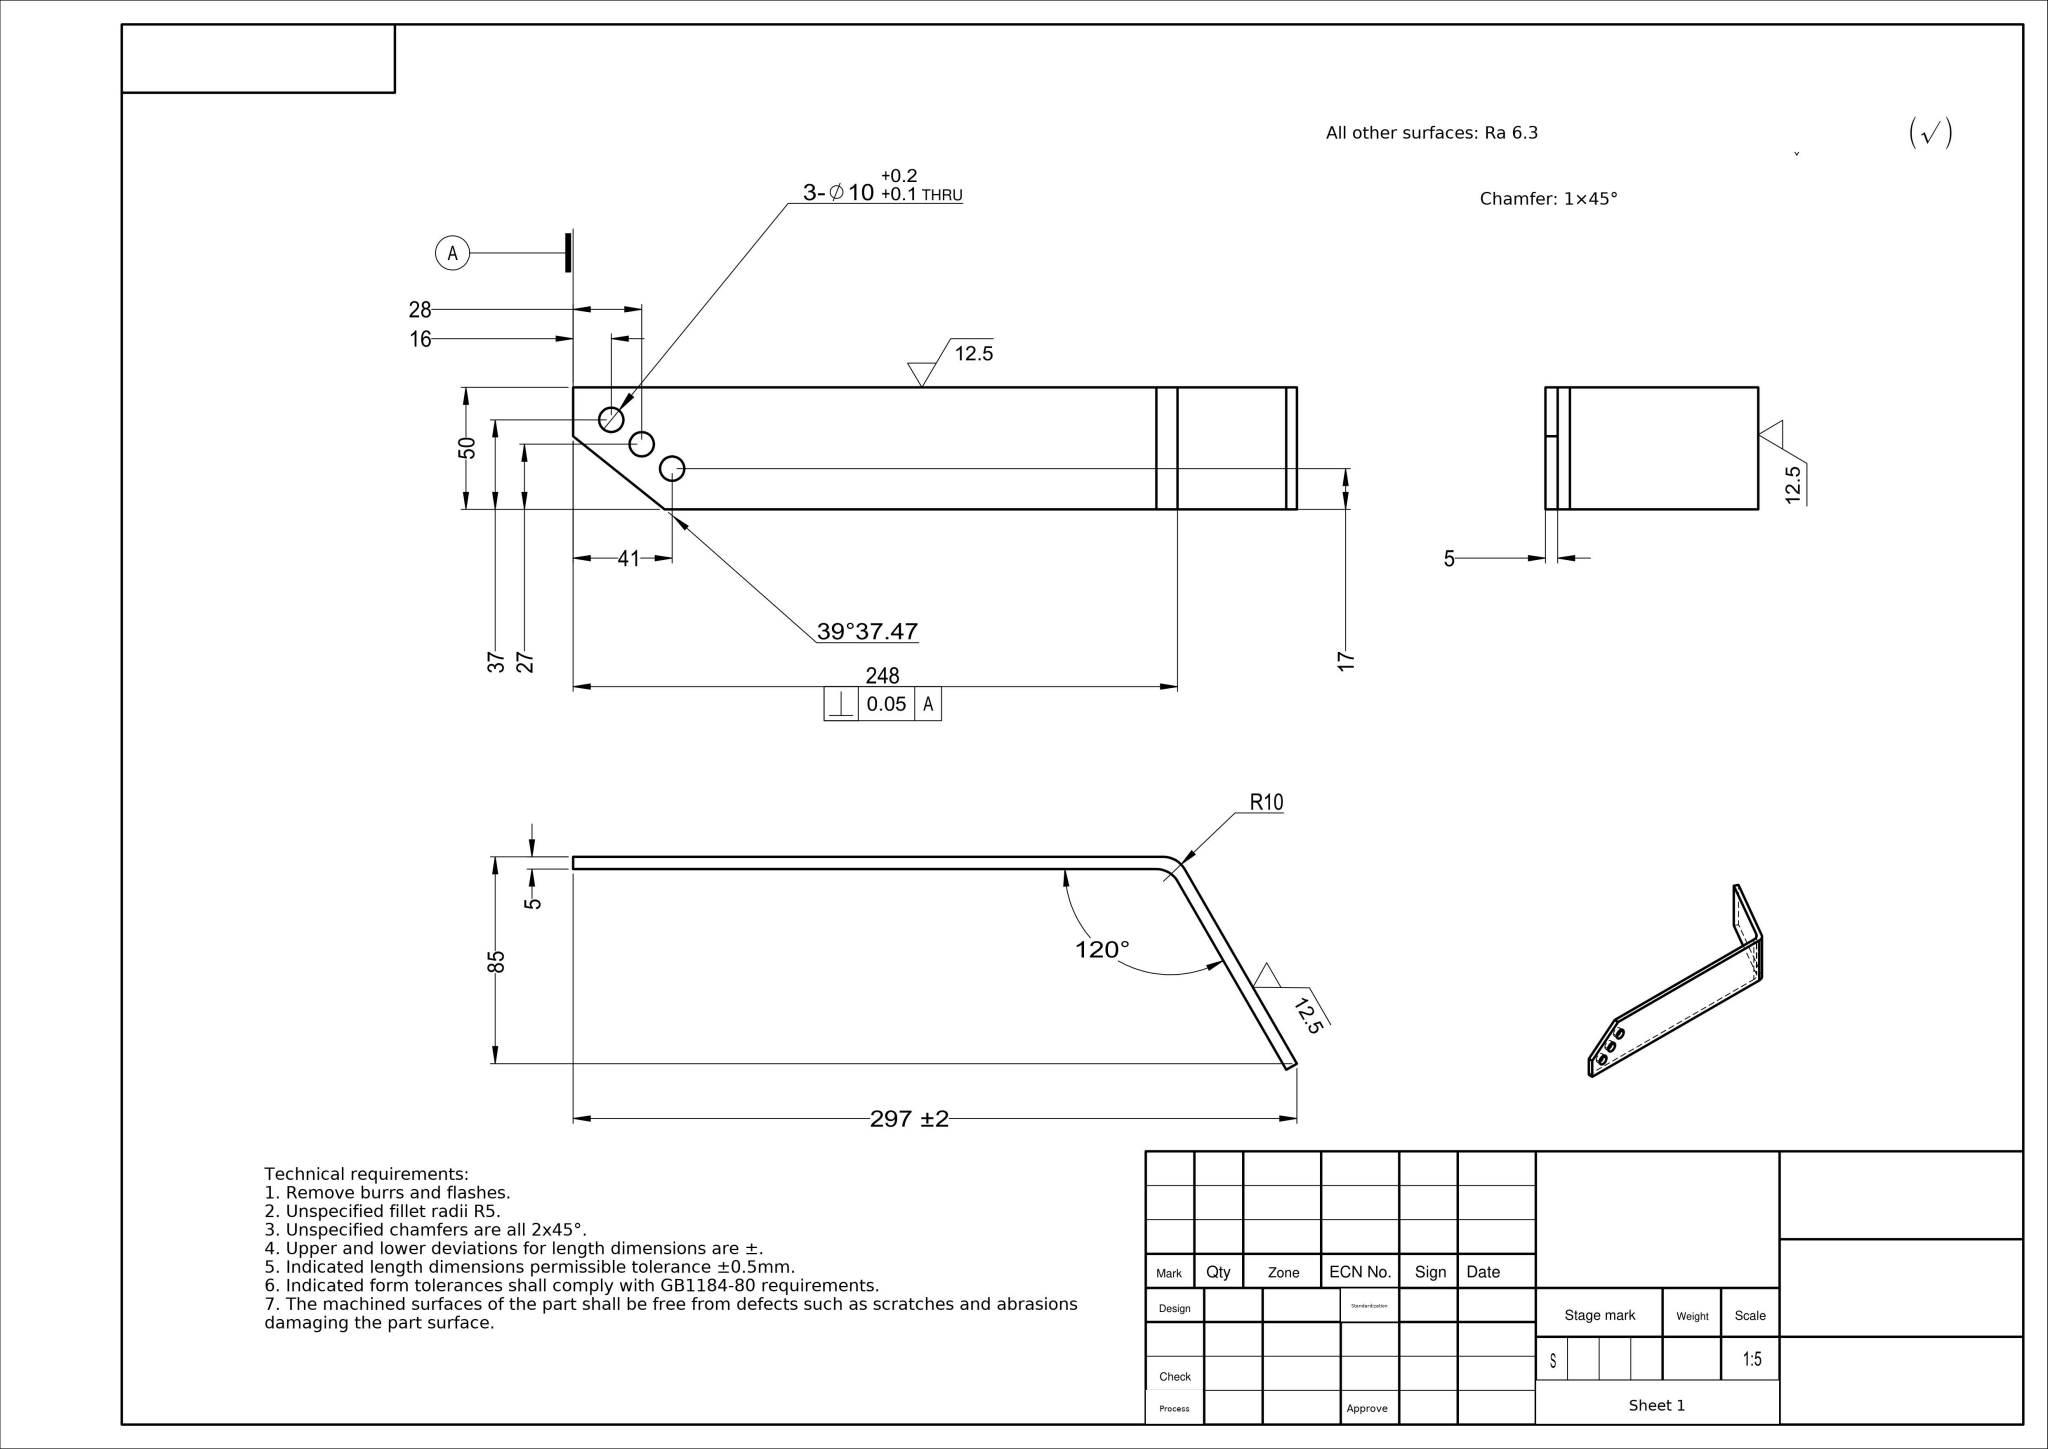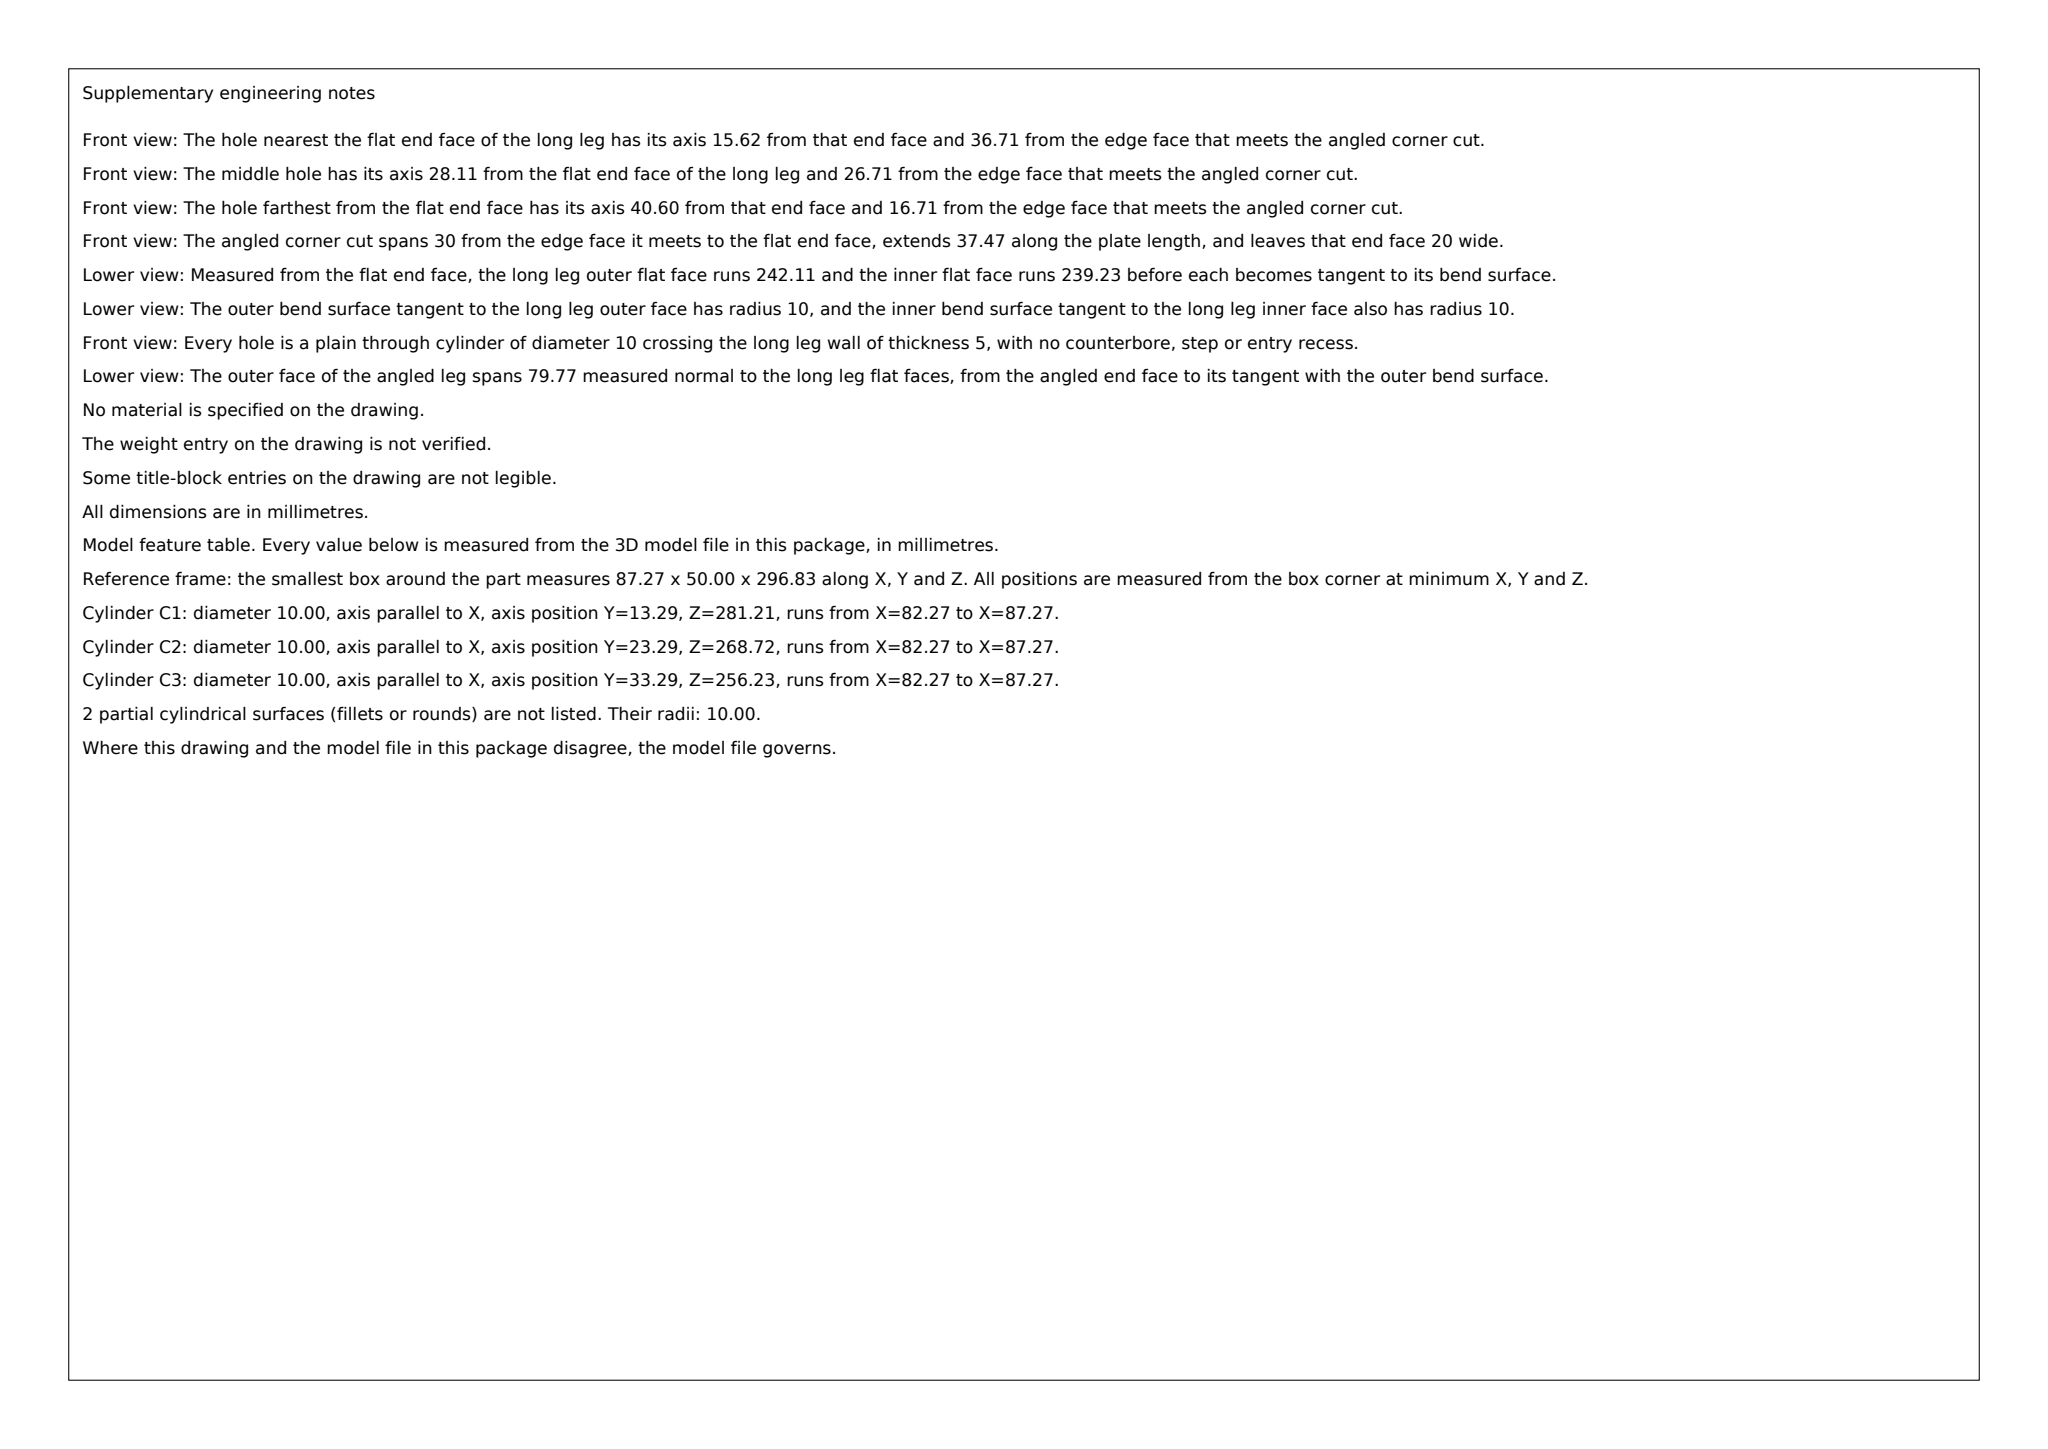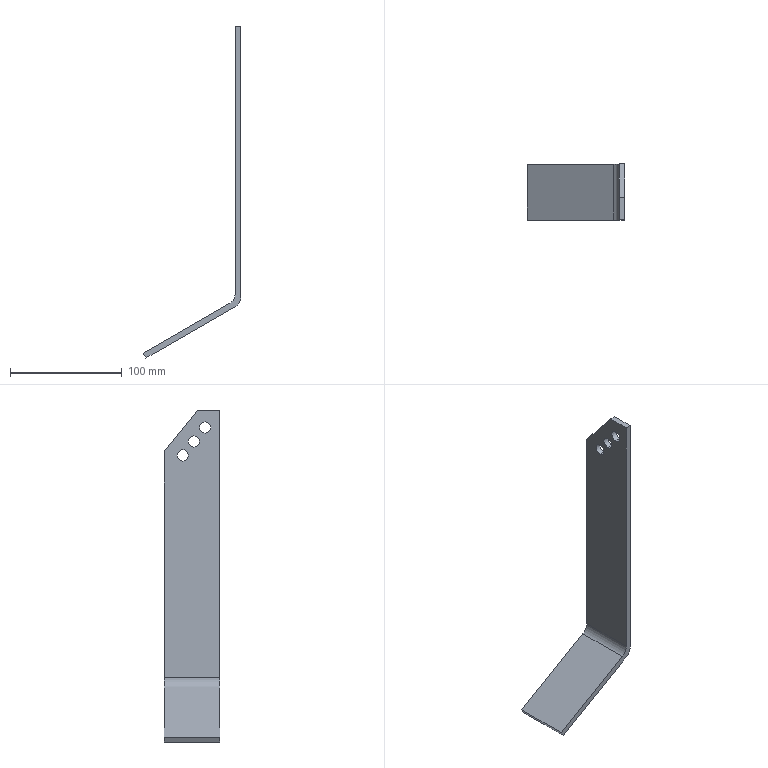Part | SolidWorks | mm | 1 solid | 17 faces | box 87.27 x 50 x 296.83 mm | volume 81733 mm3 | plane 9 | cylinder 8 | commonest cylinder face diameters 10 x6 20 x2
Drawing notes:
3X Ø10 (+0.2/+0.1) THRU holes in the 5 thick end flange, equally spaced 12.5 apart in the length direction; hole centers located 15.6, 28.1 and 40.6 from datum A (end face) | from the solid: cylinders[hole/bore, dia 10.0, axis x] at z = 281.2, 268.7, 256.2 with part end face at z = 296.8 (axis_planes z=296.8)
3X Ø10 hole centers also staggered 10 apart across the width: 13.3, 23.3 and 33.3 from the y=0 face | from the solid: cylinders[hole/bore, dia 10.0, axis x] at y = 13.3, 23.3, 33.3; axis_planes y=0.0
3X Ø10 (+0.2/+0.1) THRU holes equally spaced 12.5 apart in the length direction; hole centers at 15.6, 28.1 and 40.6 from datum A (end face). | from the solid: hole/bore Ø10 axis x at z=281.2, 268.7, 256.2 with end face plane z=296.8 (datum A); spacing 12.5, distances 15.6/28.1/40.6
STEP:
#1=CARTESIAN_POINT('',(77.272,50.,44.613));
#2=VERTEX_POINT('',#1);
#3=CARTESIAN_POINT('',(82.272,50.,53.274));
#4=VERTEX_POINT('',#3);
#5=CARTESIAN_POINT('',(72.272,50.,53.274));
#6=DIRECTION('',(0.,-1.,0.));
#7=DIRECTION('',(0.,0.,-1.));
#8=AXIS2_PLACEMENT_3D('',#5,#6,#7);
#9=CIRCLE('',#8,10.);
#10=EDGE_CURVE('',#2,#4,#9,.T.);
#11=ORIENTED_EDGE('',*,*,#10,.F.);
#12=CARTESIAN_POINT('',(77.272,0.,44.613));
#13=VERTEX_POINT('',#12);
#14=CARTESIAN_POINT('',(77.272,50.,44.613));
#15=DIRECTION('',(0.,1.,0.));
#16=VECTOR('',#15,1000.);
#17=LINE('',#14,#16);
#18=EDGE_CURVE('',#13,#2,#17,.T.);
#19=ORIENTED_EDGE('',*,*,#18,.F.);
#20=CARTESIAN_POINT('',(82.272,0.,53.274));
#21=VERTEX_POINT('',#20);
#22=CARTESIAN_POINT('',(72.272,0.,53.274));
#23=DIRECTION('',(0.,1.,0.));
#24=DIRECTION('',(0.,0.,-1.));
#25=AXIS2_PLACEMENT_3D('',#22,#23,#24);
#26=CIRCLE('',#25,10.);
#27=EDGE_CURVE('',#21,#13,#26,.T.);
#28=ORIENTED_EDGE('',*,*,#27,.F.);
#29=CARTESIAN_POINT('',(82.272,0.,53.274));
#30=DIRECTION('',(0.,-1.,0.));
#31=VECTOR('',#30,1000.);
#32=LINE('',#29,#31);
#33=EDGE_CURVE('',#4,#21,#32,.T.);
#34=ORIENTED_EDGE('',*,*,#33,.F.);
#35=EDGE_LOOP('',(#11,#19,#28,#34));
#36=FACE_OUTER_BOUND('',#35,.T.);
#37=CARTESIAN_POINT('',(72.272,50.,53.274));
#38=DIRECTION('',(0.,1.,0.));
#39=DIRECTION('',(0.,0.,1.));
#40=AXIS2_PLACEMENT_3D('',#37,#38,#39);
#41=CYLINDRICAL_SURFACE('',#40,10.);
#42=ADVANCED_FACE('',(#36),#41,.F.);
#43=CARTESIAN_POINT('',(87.272,50.,50.387));
#44=VERTEX_POINT('',#43);
#45=CARTESIAN_POINT('',(82.272,50.,41.726));
#46=VERTEX_POINT('',#45);
#47=CARTESIAN_POINT('',(77.272,50.,50.387));
#48=DIRECTION('',(0.,1.,0.));
#49=DIRECTION('',(0.,0.,-1.));
#50=AXIS2_PLACEMENT_3D('',#47,#48,#49);
#51=CIRCLE('',#50,10.);
#52=EDGE_CURVE('',#44,#46,#51,.T.);
#53=ORIENTED_EDGE('',*,*,#52,.F.);
#54=CARTESIAN_POINT('',(87.272,0.,50.387));
#55=VERTEX_POINT('',#54);
#56=CARTESIAN_POINT('',(87.272,50.,50.387));
#57=DIRECTION('',(0.,1.,0.));
#58=VECTOR('',#57,1000.);
#59=LINE('',#56,#58);
#60=EDGE_CURVE('',#55,#44,#59,.T.);
#61=ORIENTED_EDGE('',*,*,#60,.F.);
#62=CARTESIAN_POINT('',(82.272,0.,41.726));
#63=VERTEX_POINT('',#62);
#64=CARTESIAN_POINT('',(77.272,0.,50.387));
#65=DIRECTION('',(0.,-1.,0.));
#66=DIRECTION('',(0.,0.,-1.));
#67=AXIS2_PLACEMENT_3D('',#64,#65,#66);
#68=CIRCLE('',#67,10.);
#69=EDGE_CURVE('',#63,#55,#68,.T.);
#70=ORIENTED_EDGE('',*,*,#69,.F.);
#71=CARTESIAN_POINT('',(82.272,50.,41.726));
#72=DIRECTION('',(0.,-1.,0.));
#73=VECTOR('',#72,1000.);
#74=LINE('',#71,#73);
#75=EDGE_CURVE('',#46,#63,#74,.T.);
#76=ORIENTED_EDGE('',*,*,#75,.F.);
#77=EDGE_LOOP('',(#53,#61,#70,#76));
#78=FACE_OUTER_BOUND('',#77,.T.);
#79=CARTESIAN_POINT('',(77.272,50.,50.387));
#80=DIRECTION('',(0.,-1.,0.));
#81=DIRECTION('',(0.,0.,-1.));
#82=AXIS2_PLACEMENT_3D('',#79,#80,#81);
#83=CYLINDRICAL_SURFACE('',#82,10.);
#84=ADVANCED_FACE('',(#78),#83,.T.);
#85=CARTESIAN_POINT('',(82.272,13.291,281.88));
#86=VERTEX_POINT('',#85);
#87=CARTESIAN_POINT('',(87.272,13.291,281.88));
#88=VERTEX_POINT('',#87);
#89=CARTESIAN_POINT('',(37.272,13.291,281.88));
#90=DIRECTION('',(1.,0.,0.));
#91=VECTOR('',#90,1000.);
#92=LINE('',#89,#91);
#93=EDGE_CURVE('',#86,#88,#92,.T.);
#94=ORIENTED_EDGE('',*,*,#93,.F.);
#95=CARTESIAN_POINT('',(82.272,13.291,271.88));
#96=VERTEX_POINT('',#95);
#97=CARTESIAN_POINT('',(82.272,13.291,276.88));
#98=DIRECTION('',(1.,0.,0.));
#99=DIRECTION('',(0.,0.,-1.));
#100=AXIS2_PLACEMENT_3D('',#97,#98,#99);
#101=CIRCLE('',#100,5.);
#102=EDGE_CURVE('',#96,#86,#101,.T.);
#103=ORIENTED_EDGE('',*,*,#102,.F.);
#104=CARTESIAN_POINT('',(87.272,13.291,271.88));
#105=VERTEX_POINT('',#104);
#106=CARTESIAN_POINT('',(37.272,13.291,271.88));
#107=DIRECTION('',(1.,0.,0.));
#108=VECTOR('',#107,1000.);
#109=LINE('',#106,#108);
#110=EDGE_CURVE('',#96,#105,#109,.T.);
#111=ORIENTED_EDGE('',*,*,#110,.T.);
#112=CARTESIAN_POINT('',(87.272,13.291,276.88));
#113=DIRECTION('',(1.,0.,0.));
#114=DIRECTION('',(0.,0.,-1.));
#115=AXIS2_PLACEMENT_3D('',#112,#113,#114);
#116=CIRCLE('',#115,5.);
#117=EDGE_CURVE('',#105,#88,#116,.T.);
#118=ORIENTED_EDGE('',*,*,#117,.T.);
#119=EDGE_LOOP('',(#94,#103,#111,#118));
#120=FACE_OUTER_BOUND('',#119,.T.);
#121=CARTESIAN_POINT('',(37.272,13.291,276.88));
#122=DIRECTION('',(1.,0.,0.));
#123=DIRECTION('',(0.,0.,-1.));
#124=AXIS2_PLACEMENT_3D('',#121,#122,#123);
#125=CYLINDRICAL_SURFACE('',#124,5.);
#126=ADVANCED_FACE('',(#120),#125,.F.);
#127=CARTESIAN_POINT('',(82.272,33.291,256.9));
#128=VERTEX_POINT('',#127);
#129=CARTESIAN_POINT('',(87.272,33.291,256.9));
#130=VERTEX_POINT('',#129);
#131=CARTESIAN_POINT('',(37.272,33.291,256.9));
#132=DIRECTION('',(1.,0.,0.));
#133=VECTOR('',#132,1000.);
#134=LINE('',#131,#133);
#135=EDGE_CURVE('',#128,#130,#134,.T.);
#136=ORIENTED_EDGE('',*,*,#135,.F.);
#137=CARTESIAN_POINT('',(82.272,33.291,246.9));
#138=VERTEX_POINT('',#137);
#139=CARTESIAN_POINT('',(82.272,33.291,251.9));
#140=DIRECTION('',(1.,0.,0.));
#141=DIRECTION('',(0.,0.,-1.));
#142=AXIS2_PLACEMENT_3D('',#139,#140,#141);
#143=CIRCLE('',#142,5.);
#144=EDGE_CURVE('',#138,#128,#143,.T.);
#145=ORIENTED_EDGE('',*,*,#144,.F.);
#146=CARTESIAN_POINT('',(87.272,33.291,246.9));
#147=VERTEX_POINT('',#146);
#148=CARTESIAN_POINT('',(37.272,33.291,246.9));
#149=DIRECTION('',(1.,0.,0.));
#150=VECTOR('',#149,1000.);
#151=LINE('',#148,#150);
#152=EDGE_CURVE('',#138,#147,#151,.T.);
#153=ORIENTED_EDGE('',*,*,#152,.T.);
#154=CARTESIAN_POINT('',(87.272,33.291,251.9));
#155=DIRECTION('',(1.,0.,0.));
#156=DIRECTION('',(0.,0.,-1.));
#157=AXIS2_PLACEMENT_3D('',#154,#155,#156);
#158=CIRCLE('',#157,5.);
#159=EDGE_CURVE('',#147,#130,#158,.T.);
#160=ORIENTED_EDGE('',*,*,#159,.T.);
#161=EDGE_LOOP('',(#136,#145,#153,#160));
#162=FACE_OUTER_BOUND('',#161,.T.);
#163=CARTESIAN_POINT('',(37.272,33.291,251.9));
#164=DIRECTION('',(1.,0.,0.));
#165=DIRECTION('',(0.,0.,-1.));
#166=AXIS2_PLACEMENT_3D('',#163,#164,#165);
#167=CYLINDRICAL_SURFACE('',#166,5.);
#168=ADVANCED_FACE('',(#162),#167,.F.);
#169=CARTESIAN_POINT('',(82.272,23.291,269.39));
#170=VERTEX_POINT('',#169);
#171=CARTESIAN_POINT('',(87.272,23.291,269.39));
#172=VERTEX_POINT('',#171);
#173=CARTESIAN_POINT('',(37.272,23.291,269.39));
#174=DIRECTION('',(1.,0.,0.));
#175=VECTOR('',#174,1000.);
#176=LINE('',#173,#175);
#177=EDGE_CURVE('',#170,#172,#176,.T.);
#178=ORIENTED_EDGE('',*,*,#177,.F.);
#179=CARTESIAN_POINT('',(82.272,23.291,259.39));
#180=VERTEX_POINT('',#179);
#181=CARTESIAN_POINT('',(82.272,23.291,264.39));
#182=DIRECTION('',(1.,0.,0.));
#183=DIRECTION('',(0.,0.,-1.));
#184=AXIS2_PLACEMENT_3D('',#181,#182,#183);
#185=CIRCLE('',#184,5.);
#186=EDGE_CURVE('',#180,#170,#185,.T.);
#187=ORIENTED_EDGE('',*,*,#186,.F.);
#188=CARTESIAN_POINT('',(87.272,23.291,259.39));
#189=VERTEX_POINT('',#188);
#190=CARTESIAN_POINT('',(37.272,23.291,259.39));
#191=DIRECTION('',(1.,0.,0.));
#192=VECTOR('',#191,1000.);
#193=LINE('',#190,#192);
#194=EDGE_CURVE('',#180,#189,#193,.T.);
#195=ORIENTED_EDGE('',*,*,#194,.T.);
#196=CARTESIAN_POINT('',(87.272,23.291,264.39));
#197=DIRECTION('',(1.,0.,0.));
#198=DIRECTION('',(0.,0.,-1.));
#199=AXIS2_PLACEMENT_3D('',#196,#197,#198);
#200=CIRCLE('',#199,5.);
#201=EDGE_CURVE('',#189,#172,#200,.T.);
#202=ORIENTED_EDGE('',*,*,#201,.T.);
#203=EDGE_LOOP('',(#178,#187,#195,#202));
#204=FACE_OUTER_BOUND('',#203,.T.);
#205=CARTESIAN_POINT('',(37.272,23.291,264.39));
#206=DIRECTION('',(1.,0.,0.));
#207=DIRECTION('',(0.,0.,-1.));
#208=AXIS2_PLACEMENT_3D('',#205,#206,#207);
#209=CYLINDRICAL_SURFACE('',#208,5.);
#210=ADVANCED_FACE('',(#204),#209,.F.);
#211=CARTESIAN_POINT('',(82.272,20.,292.5));
#212=VERTEX_POINT('',#211);
#213=CARTESIAN_POINT('',(87.272,20.,292.5));
#214=VERTEX_POINT('',#213);
#215=CARTESIAN_POINT('',(37.272,20.,292.5));
#216=DIRECTION('',(1.,0.,0.));
#217=VECTOR('',#216,1000.);
#218=LINE('',#215,#217);
#219=EDGE_CURVE('',#212,#214,#218,.T.);
#220=ORIENTED_EDGE('',*,*,#219,.T.);
#221=CARTESIAN_POINT('',(87.272,50.,255.03));
#222=VERTEX_POINT('',#221);
#223=CARTESIAN_POINT('',(87.272,50.,255.03));
#224=DIRECTION('',(0.,0.625,-0.7806));
#225=VECTOR('',#224,1000.);
#226=LINE('',#223,#225);
#227=EDGE_CURVE('',#214,#222,#226,.T.);
#228=ORIENTED_EDGE('',*,*,#227,.T.);
#229=CARTESIAN_POINT('',(82.272,50.,255.03));
#230=VERTEX_POINT('',#229);
#231=CARTESIAN_POINT('',(0.,50.,255.03));
#232=DIRECTION('',(1.,0.,0.));
#233=VECTOR('',#232,1000.);
#234=LINE('',#231,#233);
#235=EDGE_CURVE('',#230,#222,#234,.T.);
#236=ORIENTED_EDGE('',*,*,#235,.F.);
#237=CARTESIAN_POINT('',(82.272,151.252,128.566));
#238=DIRECTION('',(-0.,0.625,-0.7806));
#239=VECTOR('',#238,1000.);
#240=LINE('',#237,#239);
#241=EDGE_CURVE('',#212,#230,#240,.T.);
#242=ORIENTED_EDGE('',*,*,#241,.F.);
#243=EDGE_LOOP('',(#220,#228,#236,#242));
#244=FACE_OUTER_BOUND('',#243,.T.);
#245=CARTESIAN_POINT('',(37.272,50.,255.03));
#246=DIRECTION('',(0.,-0.7806,-0.625));
#247=DIRECTION('',(0.,0.625,-0.7806));
#248=AXIS2_PLACEMENT_3D('',#245,#246,#247);
#249=PLANE('',#248);
#250=ADVANCED_FACE('',(#244),#249,.F.);
#251=CARTESIAN_POINT('',(2.5,0.,-4.33));
#252=VERTEX_POINT('',#251);
#253=CARTESIAN_POINT('',(2.5,0.,-4.33));
#254=DIRECTION('',(-0.866,0.,-0.5));
#255=VECTOR('',#254,1000.);
#256=LINE('',#253,#255);
#257=EDGE_CURVE('',#63,#252,#256,.T.);
#258=ORIENTED_EDGE('',*,*,#257,.F.);
#259=ORIENTED_EDGE('',*,*,#69,.T.);
#260=CARTESIAN_POINT('',(87.272,0.,292.5));
#261=VERTEX_POINT('',#260);
#262=CARTESIAN_POINT('',(87.272,0.,44.613));
#263=DIRECTION('',(-0.,0.,-1.));
#264=VECTOR('',#263,1000.);
#265=LINE('',#262,#264);
#266=EDGE_CURVE('',#261,#55,#265,.T.);
#267=ORIENTED_EDGE('',*,*,#266,.F.);
#268=CARTESIAN_POINT('',(82.272,0.,292.5));
#269=VERTEX_POINT('',#268);
#270=CARTESIAN_POINT('',(82.272,0.,292.5));
#271=DIRECTION('',(1.,0.,0.));
#272=VECTOR('',#271,1000.);
#273=LINE('',#270,#272);
#274=EDGE_CURVE('',#269,#261,#273,.T.);
#275=ORIENTED_EDGE('',*,*,#274,.F.);
#276=CARTESIAN_POINT('',(82.272,0.,47.5));
#277=DIRECTION('',(0.,0.,1.));
#278=VECTOR('',#277,1000.);
#279=LINE('',#276,#278);
#280=EDGE_CURVE('',#21,#269,#279,.T.);
#281=ORIENTED_EDGE('',*,*,#280,.F.);
#282=ORIENTED_EDGE('',*,*,#27,.T.);
#283=CARTESIAN_POINT('',(0.,0.,0.));
#284=VERTEX_POINT('',#283);
#285=CARTESIAN_POINT('',(0.,0.,0.));
#286=DIRECTION('',(0.866,0.,0.5));
#287=VECTOR('',#286,1000.);
#288=LINE('',#285,#287);
#289=EDGE_CURVE('',#284,#13,#288,.T.);
#290=ORIENTED_EDGE('',*,*,#289,.F.);
#291=CARTESIAN_POINT('',(0.,0.,0.));
#292=DIRECTION('',(-0.5,0.,0.866));
#293=VECTOR('',#292,1000.);
#294=LINE('',#291,#293);
#295=EDGE_CURVE('',#252,#284,#294,.T.);
#296=ORIENTED_EDGE('',*,*,#295,.F.);
#297=EDGE_LOOP('',(#258,#259,#267,#275,#281,#282,#290,#296));
#298=FACE_OUTER_BOUND('',#297,.T.);
#299=CARTESIAN_POINT('',(0.,0.,0.));
#300=DIRECTION('',(0.,-1.,0.));
#301=DIRECTION('',(0.,0.,-1.));
#302=AXIS2_PLACEMENT_3D('',#299,#300,#301);
#303=PLANE('',#302);
#304=ADVANCED_FACE('',(#298),#303,.T.);
#305=CARTESIAN_POINT('',(87.272,50.,44.613));
#306=DIRECTION('',(-0.,0.,-1.));
#307=VECTOR('',#306,1000.);
#308=LINE('',#305,#307);
#309=EDGE_CURVE('',#222,#44,#308,.T.);
#310=ORIENTED_EDGE('',*,*,#309,.T.);
#311=ORIENTED_EDGE('',*,*,#52,.T.);
#312=CARTESIAN_POINT('',(2.5,50.,-4.33));
#313=VERTEX_POINT('',#312);
#314=CARTESIAN_POINT('',(2.5,50.,-4.33));
#315=DIRECTION('',(-0.866,0.,-0.5));
#316=VECTOR('',#315,1000.);
#317=LINE('',#314,#316);
#318=EDGE_CURVE('',#46,#313,#317,.T.);
#319=ORIENTED_EDGE('',*,*,#318,.T.);
#320=CARTESIAN_POINT('',(0.,50.,0.));
#321=VERTEX_POINT('',#320);
#322=CARTESIAN_POINT('',(0.,50.,0.));
#323=DIRECTION('',(-0.5,0.,0.866));
#324=VECTOR('',#323,1000.);
#325=LINE('',#322,#324);
#326=EDGE_CURVE('',#313,#321,#325,.T.);
#327=ORIENTED_EDGE('',*,*,#326,.T.);
#328=CARTESIAN_POINT('',(0.,50.,0.));
#329=DIRECTION('',(0.866,0.,0.5));
#330=VECTOR('',#329,1000.);
#331=LINE('',#328,#330);
#332=EDGE_CURVE('',#321,#2,#331,.T.);
#333=ORIENTED_EDGE('',*,*,#332,.T.);
#334=ORIENTED_EDGE('',*,*,#10,.T.);
#335=CARTESIAN_POINT('',(82.272,50.,47.5));
#336=DIRECTION('',(0.,0.,1.));
#337=VECTOR('',#336,1000.);
#338=LINE('',#335,#337);
#339=EDGE_CURVE('',#4,#230,#338,.T.);
#340=ORIENTED_EDGE('',*,*,#339,.T.);
#341=ORIENTED_EDGE('',*,*,#235,.T.);
#342=EDGE_LOOP('',(#310,#311,#319,#327,#333,#334,#340,#341));
#343=FACE_OUTER_BOUND('',#342,.T.);
#344=CARTESIAN_POINT('',(0.,50.,0.));
#345=DIRECTION('',(0.,-1.,0.));
#346=DIRECTION('',(0.,0.,-1.));
#347=AXIS2_PLACEMENT_3D('',#344,#345,#346);
#348=PLANE('',#347);
#349=ADVANCED_FACE('',(#343),#348,.F.);
#350=ORIENTED_EDGE('',*,*,#318,.F.);
#351=ORIENTED_EDGE('',*,*,#75,.T.);
#352=ORIENTED_EDGE('',*,*,#257,.T.);
#353=CARTESIAN_POINT('',(2.5,50.,-4.33));
#354=DIRECTION('',(0.,-1.,0.));
#355=VECTOR('',#354,1000.);
#356=LINE('',#353,#355);
#357=EDGE_CURVE('',#313,#252,#356,.T.);
#358=ORIENTED_EDGE('',*,*,#357,.F.);
#359=EDGE_LOOP('',(#350,#351,#352,#358));
#360=FACE_OUTER_BOUND('',#359,.T.);
#361=CARTESIAN_POINT('',(2.5,50.,-4.33));
#362=DIRECTION('',(-0.5,0.,0.866));
#363=DIRECTION('',(0.,1.,0.));
#364=AXIS2_PLACEMENT_3D('',#361,#362,#363);
#365=PLANE('',#364);
#366=ADVANCED_FACE('',(#360),#365,.F.);
#367=ORIENTED_EDGE('',*,*,#201,.F.);
#368=CARTESIAN_POINT('',(87.272,23.291,264.39));
#369=DIRECTION('',(1.,0.,0.));
#370=DIRECTION('',(0.,0.,-1.));
#371=AXIS2_PLACEMENT_3D('',#368,#369,#370);
#372=CIRCLE('',#371,5.);
#373=EDGE_CURVE('',#172,#189,#372,.T.);
#374=ORIENTED_EDGE('',*,*,#373,.F.);
#375=EDGE_LOOP('',(#367,#374));
#376=FACE_BOUND('',#375,.T.);
#377=ORIENTED_EDGE('',*,*,#159,.F.);
#378=CARTESIAN_POINT('',(87.272,33.291,251.9));
#379=DIRECTION('',(1.,0.,0.));
#380=DIRECTION('',(0.,0.,-1.));
#381=AXIS2_PLACEMENT_3D('',#378,#379,#380);
#382=CIRCLE('',#381,5.);
#383=EDGE_CURVE('',#130,#147,#382,.T.);
#384=ORIENTED_EDGE('',*,*,#383,.F.);
#385=EDGE_LOOP('',(#377,#384));
#386=FACE_BOUND('',#385,.T.);
#387=ORIENTED_EDGE('',*,*,#117,.F.);
#388=CARTESIAN_POINT('',(87.272,13.291,276.88));
#389=DIRECTION('',(1.,0.,0.));
#390=DIRECTION('',(0.,0.,-1.));
#391=AXIS2_PLACEMENT_3D('',#388,#389,#390);
#392=CIRCLE('',#391,5.);
#393=EDGE_CURVE('',#88,#105,#392,.T.);
#394=ORIENTED_EDGE('',*,*,#393,.F.);
#395=EDGE_LOOP('',(#387,#394));
#396=FACE_BOUND('',#395,.T.);
#397=ORIENTED_EDGE('',*,*,#266,.T.);
#398=ORIENTED_EDGE('',*,*,#60,.T.);
#399=ORIENTED_EDGE('',*,*,#309,.F.);
#400=ORIENTED_EDGE('',*,*,#227,.F.);
#401=CARTESIAN_POINT('',(87.272,50.,292.5));
#402=DIRECTION('',(0.,-1.,0.));
#403=VECTOR('',#402,1000.);
#404=LINE('',#401,#403);
#405=EDGE_CURVE('',#214,#261,#404,.T.);
#406=ORIENTED_EDGE('',*,*,#405,.T.);
#407=EDGE_LOOP('',(#397,#398,#399,#400,#406));
#408=FACE_OUTER_BOUND('',#407,.T.);
#409=CARTESIAN_POINT('',(87.272,50.,44.613));
#410=DIRECTION('',(-1.,0.,0.));
#411=DIRECTION('',(0.,1.,0.));
#412=AXIS2_PLACEMENT_3D('',#409,#410,#411);
#413=PLANE('',#412);
#414=ADVANCED_FACE('',(#376,#386,#396,#408),#413,.F.);
#415=ORIENTED_EDGE('',*,*,#405,.F.);
#416=ORIENTED_EDGE('',*,*,#219,.F.);
#417=CARTESIAN_POINT('',(82.272,50.,292.5));
#418=DIRECTION('',(0.,-1.,0.));
#419=VECTOR('',#418,1000.);
#420=LINE('',#417,#419);
#421=EDGE_CURVE('',#212,#269,#420,.T.);
#422=ORIENTED_EDGE('',*,*,#421,.T.);
#423=ORIENTED_EDGE('',*,*,#274,.T.);
#424=EDGE_LOOP('',(#415,#416,#422,#423));
#425=FACE_OUTER_BOUND('',#424,.T.);
#426=CARTESIAN_POINT('',(82.272,50.,292.5));
#427=DIRECTION('',(0.,0.,-1.));
#428=DIRECTION('',(0.,-1.,0.));
#429=AXIS2_PLACEMENT_3D('',#426,#427,#428);
#430=PLANE('',#429);
#431=ADVANCED_FACE('',(#425),#430,.F.);
#432=ORIENTED_EDGE('',*,*,#186,.T.);
#433=CARTESIAN_POINT('',(82.272,23.291,264.39));
#434=DIRECTION('',(1.,0.,0.));
#435=DIRECTION('',(0.,0.,-1.));
#436=AXIS2_PLACEMENT_3D('',#433,#434,#435);
#437=CIRCLE('',#436,5.);
#438=EDGE_CURVE('',#170,#180,#437,.T.);
#439=ORIENTED_EDGE('',*,*,#438,.T.);
#440=EDGE_LOOP('',(#432,#439));
#441=FACE_BOUND('',#440,.T.);
#442=ORIENTED_EDGE('',*,*,#144,.T.);
#443=CARTESIAN_POINT('',(82.272,33.291,251.9));
#444=DIRECTION('',(1.,0.,0.));
#445=DIRECTION('',(0.,0.,-1.));
#446=AXIS2_PLACEMENT_3D('',#443,#444,#445);
#447=CIRCLE('',#446,5.);
#448=EDGE_CURVE('',#128,#138,#447,.T.);
#449=ORIENTED_EDGE('',*,*,#448,.T.);
#450=EDGE_LOOP('',(#442,#449));
#451=FACE_BOUND('',#450,.T.);
#452=ORIENTED_EDGE('',*,*,#102,.T.);
#453=CARTESIAN_POINT('',(82.272,13.291,276.88));
#454=DIRECTION('',(1.,0.,0.));
#455=DIRECTION('',(0.,0.,-1.));
#456=AXIS2_PLACEMENT_3D('',#453,#454,#455);
#457=CIRCLE('',#456,5.);
#458=EDGE_CURVE('',#86,#96,#457,.T.);
#459=ORIENTED_EDGE('',*,*,#458,.T.);
#460=EDGE_LOOP('',(#452,#459));
#461=FACE_BOUND('',#460,.T.);
#462=ORIENTED_EDGE('',*,*,#339,.F.);
#463=ORIENTED_EDGE('',*,*,#33,.T.);
#464=ORIENTED_EDGE('',*,*,#280,.T.);
#465=ORIENTED_EDGE('',*,*,#421,.F.);
#466=ORIENTED_EDGE('',*,*,#241,.T.);
#467=EDGE_LOOP('',(#462,#463,#464,#465,#466));
#468=FACE_OUTER_BOUND('',#467,.T.);
#469=CARTESIAN_POINT('',(82.272,50.,47.5));
#470=DIRECTION('',(1.,0.,-0.));
#471=DIRECTION('',(-0.,0.,-1.));
#472=AXIS2_PLACEMENT_3D('',#469,#470,#471);
#473=PLANE('',#472);
#474=ADVANCED_FACE('',(#441,#451,#461,#468),#473,.F.);
#475=ORIENTED_EDGE('',*,*,#289,.T.);
#476=ORIENTED_EDGE('',*,*,#18,.T.);
#477=ORIENTED_EDGE('',*,*,#332,.F.);
#478=CARTESIAN_POINT('',(0.,50.,0.));
#479=DIRECTION('',(0.,-1.,0.));
#480=VECTOR('',#479,1000.);
#481=LINE('',#478,#480);
#482=EDGE_CURVE('',#321,#284,#481,.T.);
#483=ORIENTED_EDGE('',*,*,#482,.T.);
#484=EDGE_LOOP('',(#475,#476,#477,#483));
#485=FACE_OUTER_BOUND('',#484,.T.);
#486=CARTESIAN_POINT('',(0.,50.,0.));
#487=DIRECTION('',(0.5,0.,-0.866));
#488=DIRECTION('',(0.,-1.,0.));
#489=AXIS2_PLACEMENT_3D('',#486,#487,#488);
#490=PLANE('',#489);
#491=ADVANCED_FACE('',(#485),#490,.F.);
#492=ORIENTED_EDGE('',*,*,#295,.T.);
#493=ORIENTED_EDGE('',*,*,#482,.F.);
#494=ORIENTED_EDGE('',*,*,#326,.F.);
#495=ORIENTED_EDGE('',*,*,#357,.T.);
#496=EDGE_LOOP('',(#492,#493,#494,#495));
#497=FACE_OUTER_BOUND('',#496,.T.);
#498=CARTESIAN_POINT('',(0.,50.,0.));
#499=DIRECTION('',(0.866,0.,0.5));
#500=DIRECTION('',(0.,-1.,0.));
#501=AXIS2_PLACEMENT_3D('',#498,#499,#500);
#502=PLANE('',#501);
#503=ADVANCED_FACE('',(#497),#502,.F.);
#504=ORIENTED_EDGE('',*,*,#438,.F.);
#505=ORIENTED_EDGE('',*,*,#177,.T.);
#506=ORIENTED_EDGE('',*,*,#373,.T.);
#507=ORIENTED_EDGE('',*,*,#194,.F.);
#508=EDGE_LOOP('',(#504,#505,#506,#507));
#509=FACE_OUTER_BOUND('',#508,.T.);
#510=CARTESIAN_POINT('',(37.272,23.291,264.39));
#511=DIRECTION('',(1.,0.,0.));
#512=DIRECTION('',(0.,0.,-1.));
#513=AXIS2_PLACEMENT_3D('',#510,#511,#512);
#514=CYLINDRICAL_SURFACE('',#513,5.);
#515=ADVANCED_FACE('',(#509),#514,.F.);
#516=ORIENTED_EDGE('',*,*,#448,.F.);
#517=ORIENTED_EDGE('',*,*,#135,.T.);
#518=ORIENTED_EDGE('',*,*,#383,.T.);
#519=ORIENTED_EDGE('',*,*,#152,.F.);
#520=EDGE_LOOP('',(#516,#517,#518,#519));
#521=FACE_OUTER_BOUND('',#520,.T.);
#522=CARTESIAN_POINT('',(37.272,33.291,251.9));
#523=DIRECTION('',(1.,0.,0.));
#524=DIRECTION('',(0.,0.,-1.));
#525=AXIS2_PLACEMENT_3D('',#522,#523,#524);
#526=CYLINDRICAL_SURFACE('',#525,5.);
#527=ADVANCED_FACE('',(#521),#526,.F.);
#528=ORIENTED_EDGE('',*,*,#458,.F.);
#529=ORIENTED_EDGE('',*,*,#93,.T.);
#530=ORIENTED_EDGE('',*,*,#393,.T.);
#531=ORIENTED_EDGE('',*,*,#110,.F.);
#532=EDGE_LOOP('',(#528,#529,#530,#531));
#533=FACE_OUTER_BOUND('',#532,.T.);
#534=CARTESIAN_POINT('',(37.272,13.291,276.88));
#535=DIRECTION('',(1.,0.,0.));
#536=DIRECTION('',(0.,0.,-1.));
#537=AXIS2_PLACEMENT_3D('',#534,#535,#536);
#538=CYLINDRICAL_SURFACE('',#537,5.);
#539=ADVANCED_FACE('',(#533),#538,.F.);
#540=CLOSED_SHELL('',(#42,#84,#126,#168,#210,#250,#304,#349,#366,#414,#431,#474,#491,#503,#515,#527,#539));
#541=MANIFOLD_SOLID_BREP('',#540);
#542=CARTESIAN_POINT('',(0.,0.,0.));
#543=DIRECTION('',(0.,0.,1.));
#544=DIRECTION('',(1.,0.,0.));
#545=AXIS2_PLACEMENT_3D('',#542,#543,#544);
#546=(LENGTH_UNIT()NAMED_UNIT(*)SI_UNIT(.MILLI.,.METRE.));
#547=UNCERTAINTY_MEASURE_WITH_UNIT(LENGTH_MEASURE(0.00001),#546,'','');
#548=(NAMED_UNIT(*)PLANE_ANGLE_UNIT()SI_UNIT($,.RADIAN.));
#549=(NAMED_UNIT(*)SI_UNIT($,.STERADIAN.)SOLID_ANGLE_UNIT());
#550=(GEOMETRIC_REPRESENTATION_CONTEXT(3)GLOBAL_UNCERTAINTY_ASSIGNED_CONTEXT((#547))GLOBAL_UNIT_ASSIGNED_CONTEXT((#546,#548,#549))REPRESENTATION_CONTEXT('',''));
#551=ADVANCED_BREP_SHAPE_REPRESENTATION('',(#541,#545),#550);